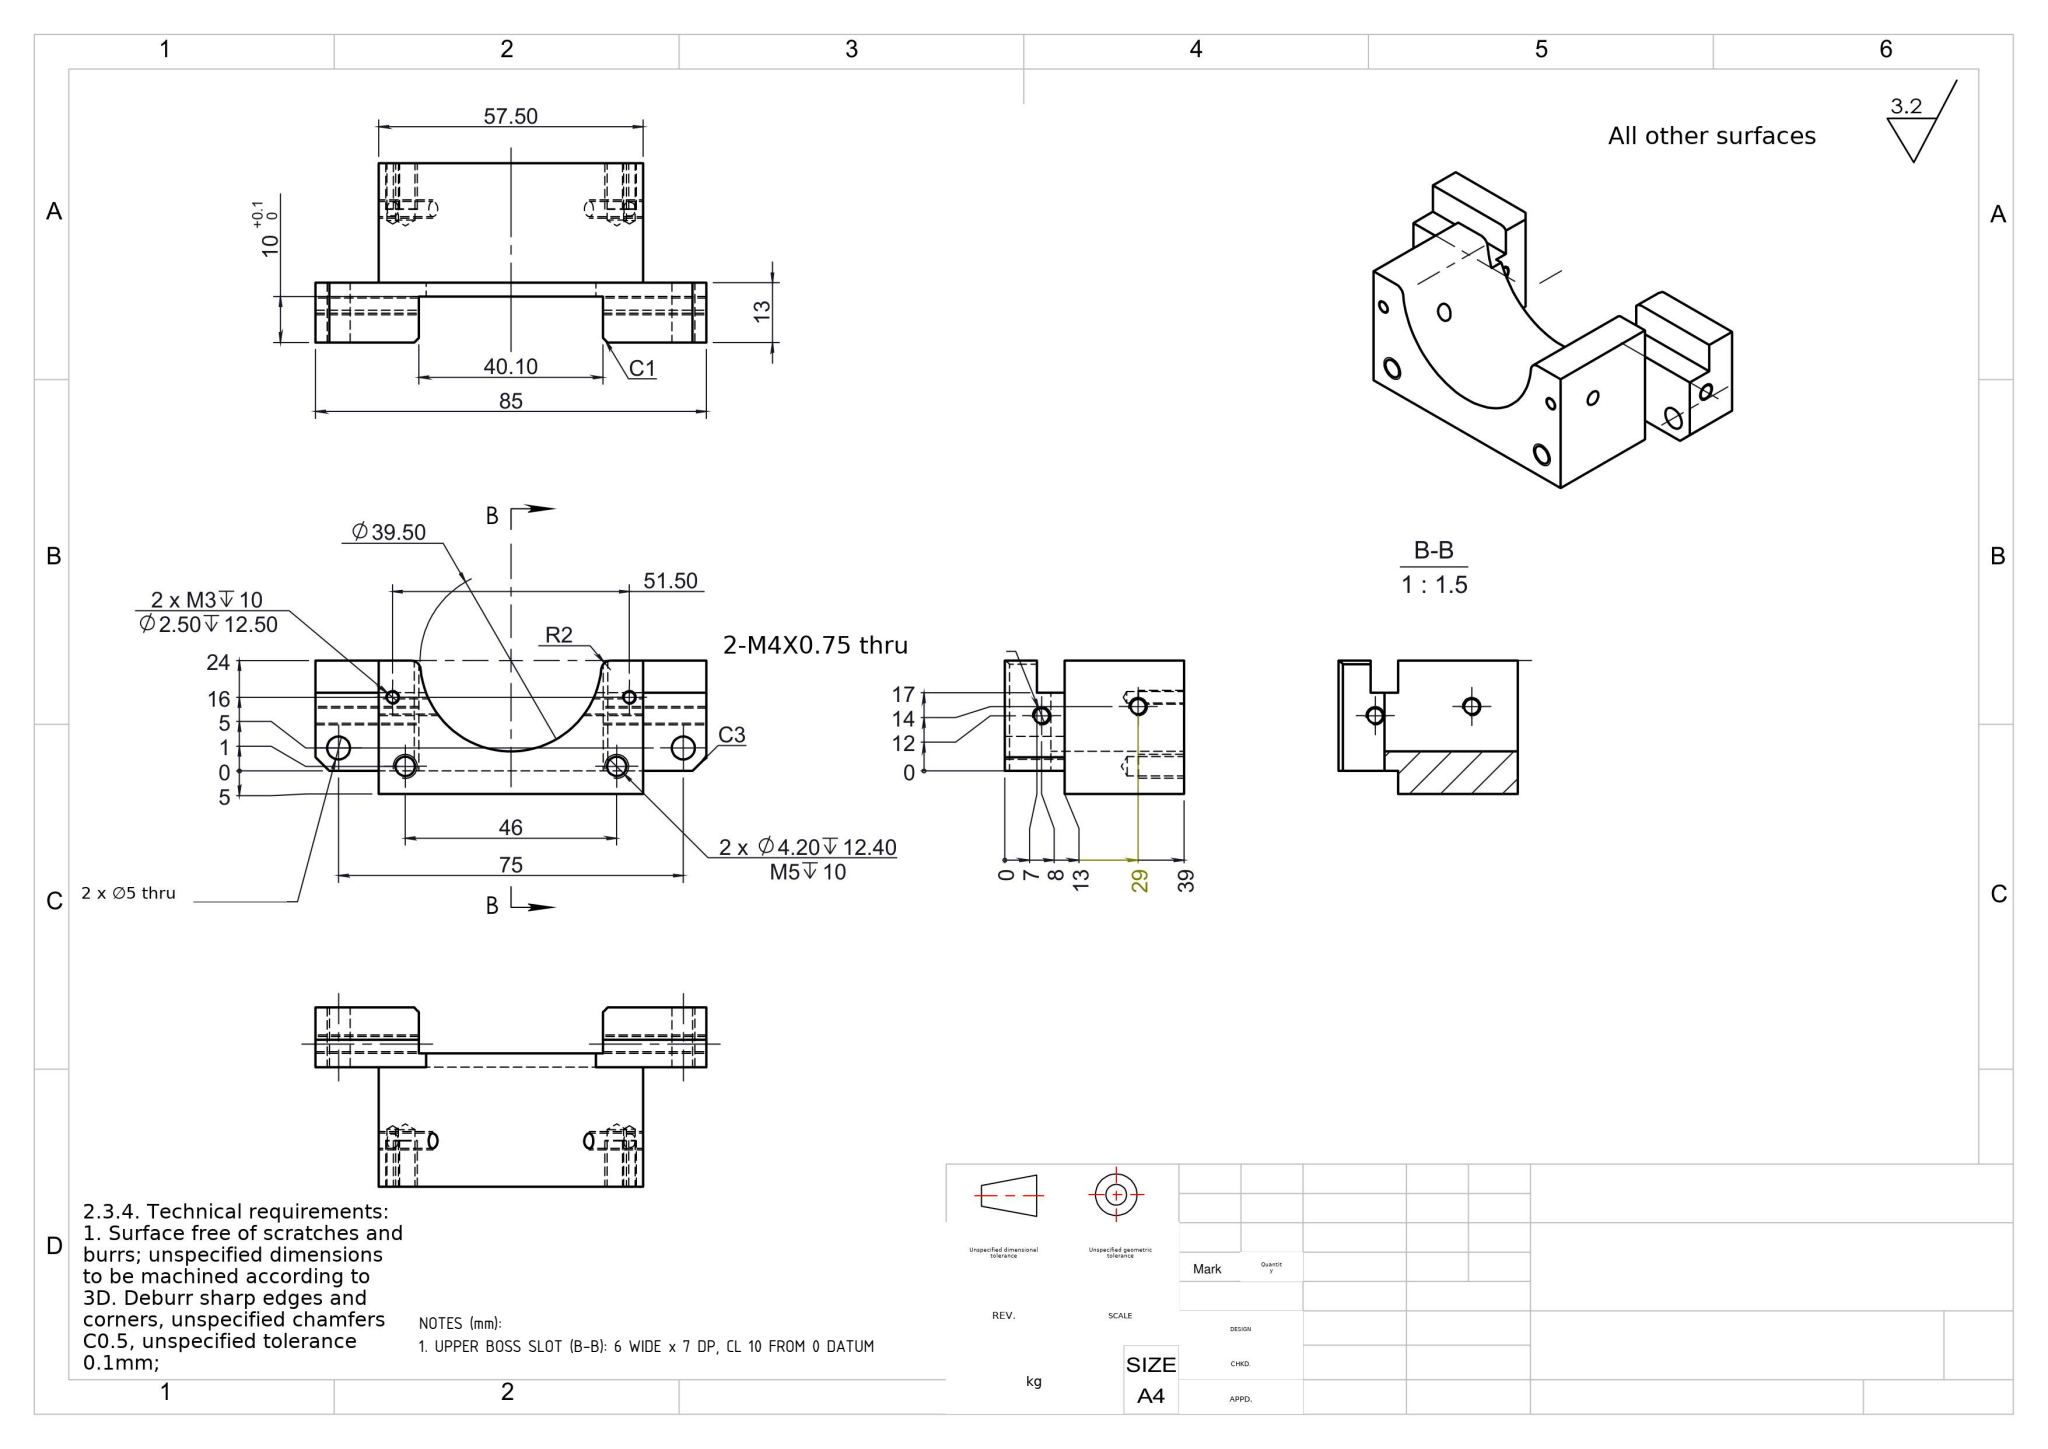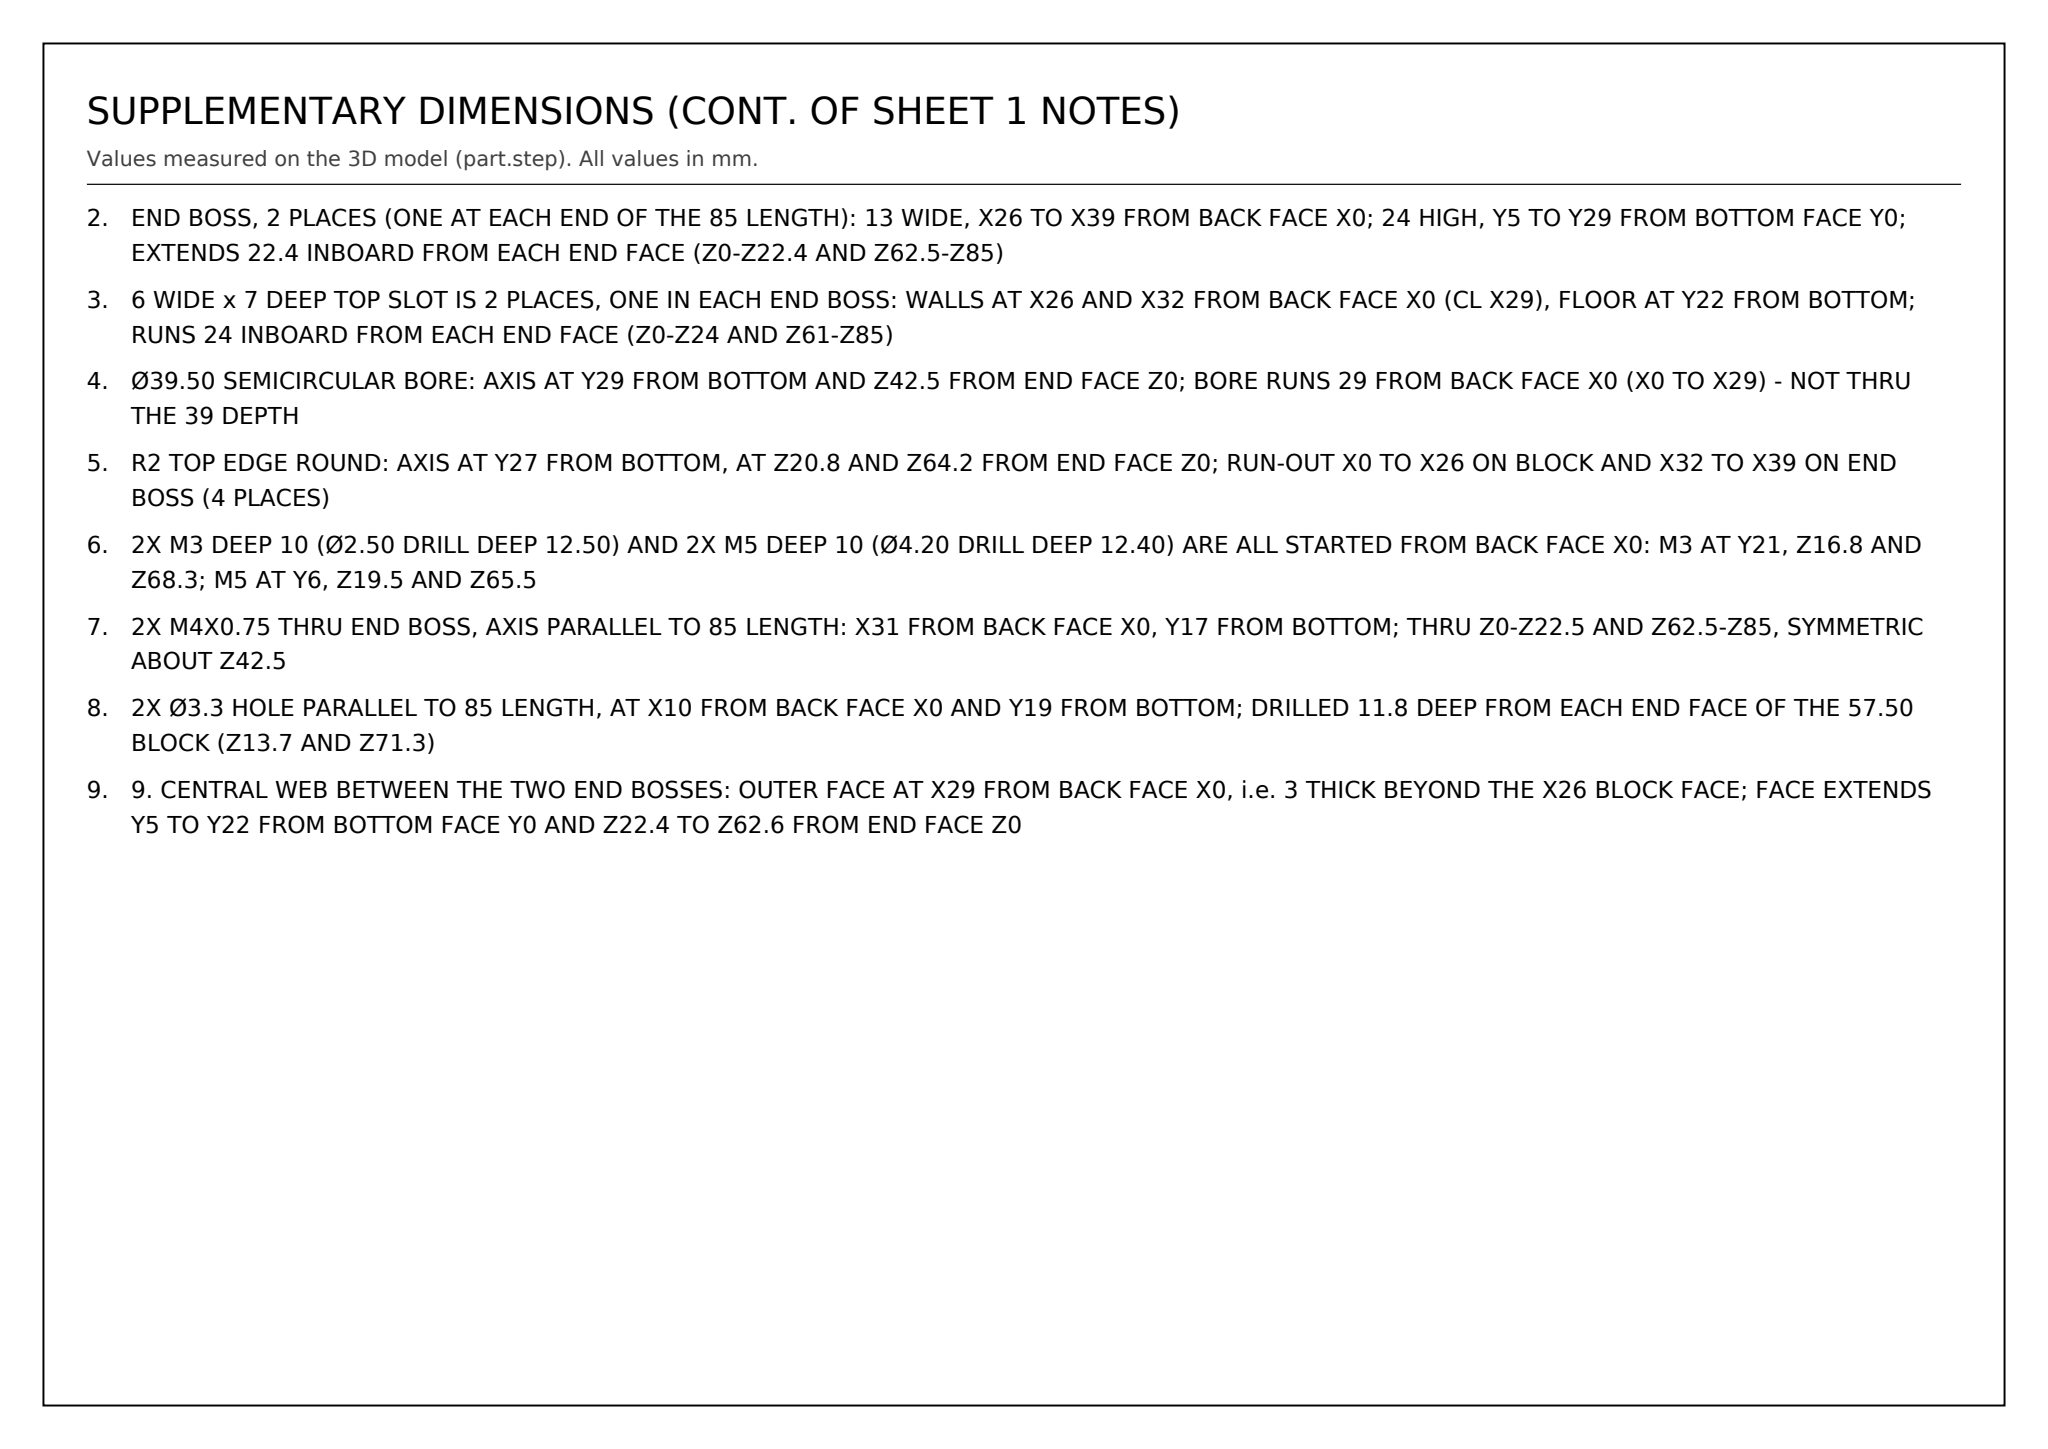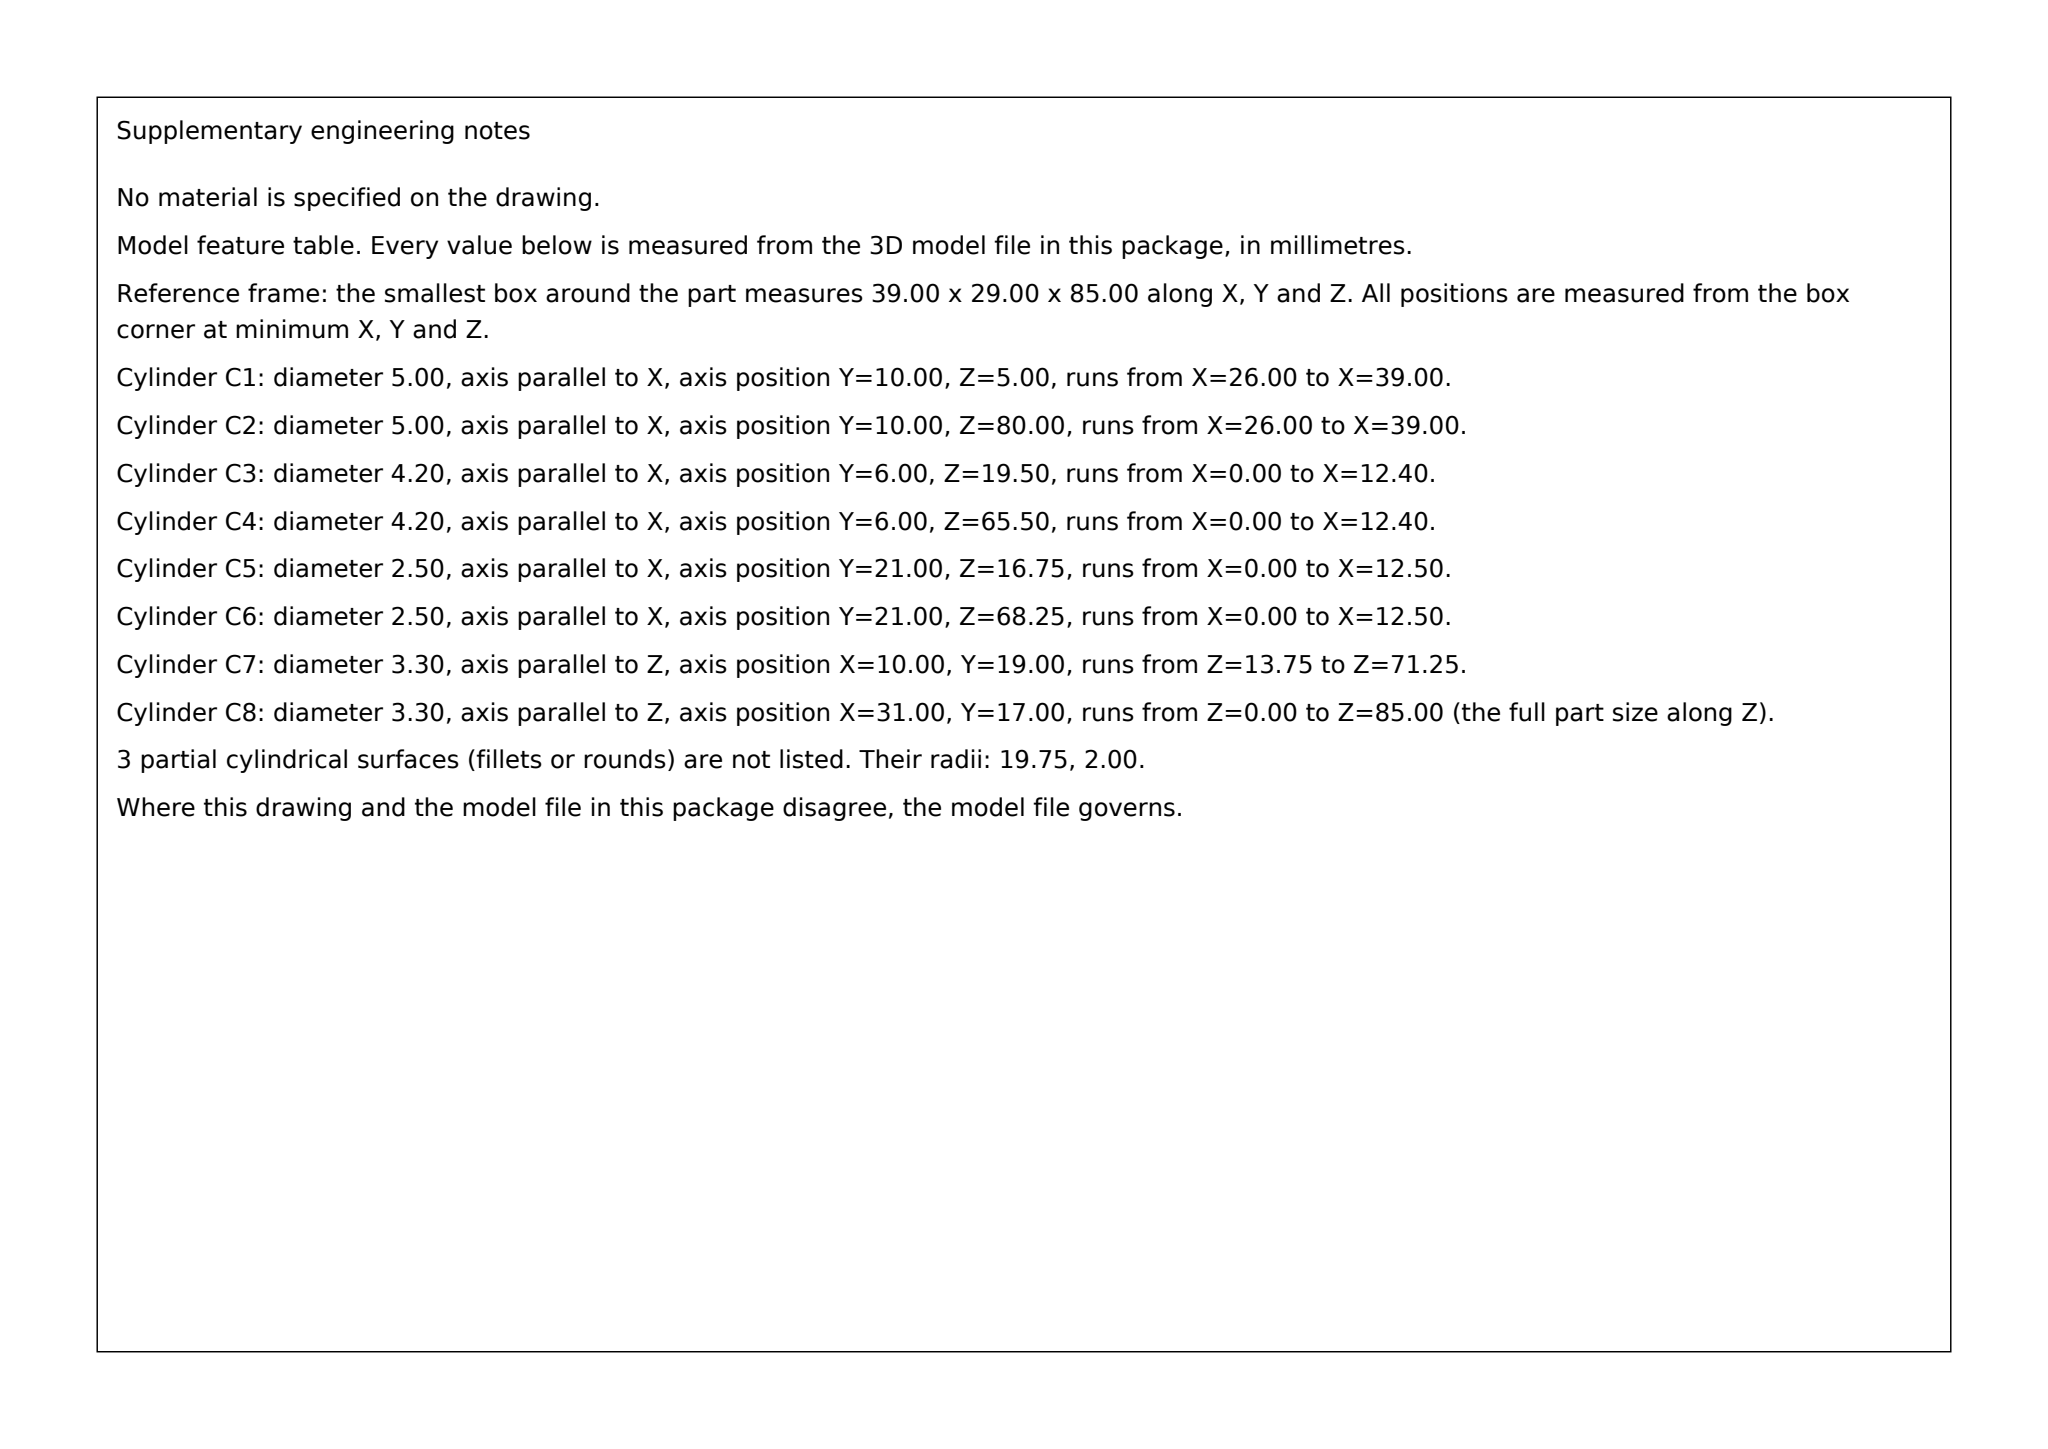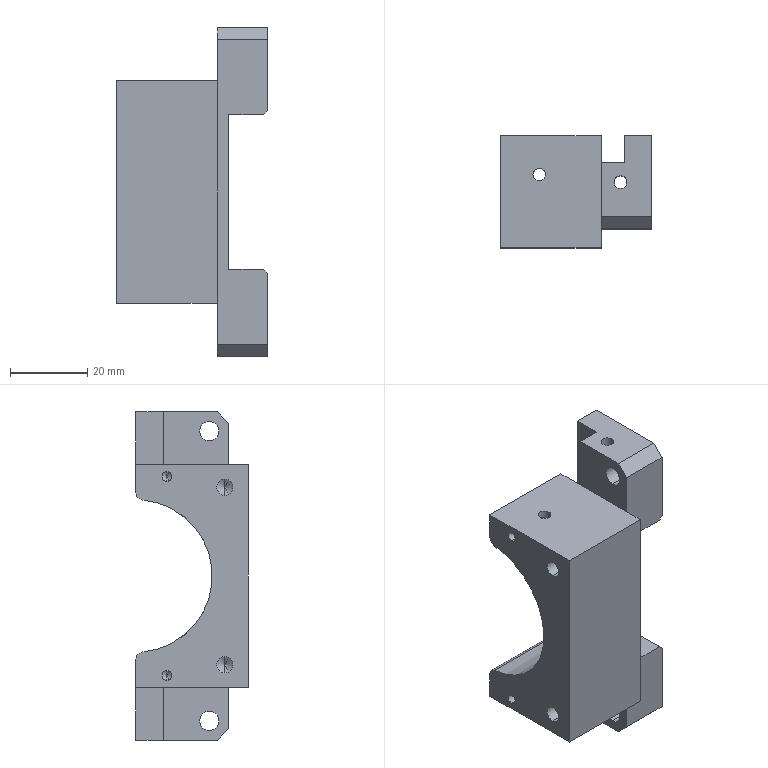Part | SolidWorks | mm | 1 solid | 62 faces | box 39 x 29 x 85 mm | volume 38812 mm3 | plane 29 | cylinder 25 | cone 8 | commonest cylinder face diameters 3.3 x8 4.2 x4 2.5 x4 5 x4 4 x4 39.5 x1
Drawing notes:
UPPER BOSS SLOT (B-B): 6 WIDE x 7 DP, CL 10 FROM 0 DATUM | from the solid: M4 x-holes split into 7 + 26 lg segments over 39 bbox -> gap x=7..13 (6 wide, CL x=10); y-planes 22 (2 slot floors) vs 29 (4 boss tops) -> 7 deep
END BOSS, 2 PLACES (ONE AT EACH END OF THE 85 LENGTH): 13 WIDE, X26 TO X39 FROM BACK FACE X0; 24 HIGH, Y5 TO Y29 FROM BOTTOM FACE Y0; EXTENDS 22.4 INBOARD FROM EACH END FACE (Z0-Z22.4 AND Z62.5-Z85) | from the solid: axis_planes x=26 / x=32 / x=39 (y 5-29), y=5 (x 26-39, z 3-82), z=22.4 and z=62.5 (x 29-38, y 5-28.2)
6 WIDE x 7 DEEP TOP SLOT IS 2 PLACES, ONE IN EACH END BOSS: WALLS AT X26 AND X32 FROM BACK FACE X0 (CL X29), FLOOR AT Y22 FROM BOTTOM; RUNS 24 INBOARD FROM EACH END FACE (Z0-Z24 AND Z61-Z85) | from the solid: axis_planes y=22, extent x 26-32, z 0-24 and z 61-85; planes x=26 and x=32 (y 22-29)
Ø39.50 SEMICIRCULAR BORE: AXIS AT Y29 FROM BOTTOM AND Z42.5 FROM END FACE Z0; BORE RUNS 29 FROM BACK FACE X0 (X0 TO X29) - NOT THRU THE 39 DEPTH | from the solid: cylinder concave arc Ø39.5, axis x, axis_pos y=29 z=42.5, from x 0.0 to 29.0, 169 deg
R2 TOP EDGE ROUND: AXIS AT Y27 FROM BOTTOM, AT Z20.8 AND Z64.2 FROM END FACE Z0; RUN-OUT X0 TO X26 ON BLOCK AND X32 TO X39 ON END BOSS (4 PLACES) | from the solid: convex arcs Ø4.0, axis x, at (y27,z20.8) and (y27,z64.2), from x 0-26 and x 32-39
2X M3 DEEP 10 (Ø2.50 DRILL DEEP 12.50) AND 2X M5 DEEP 10 (Ø4.20 DRILL DEEP 12.40) ARE ALL STARTED FROM BACK FACE X0: M3 AT Y21, Z16.8 AND Z68.3; M5 AT Y6, Z19.5 AND Z65.5 | from the solid: holes Ø2.5 axis x at (y21, z16.8/z68.3) from x0 to 12.5; holes Ø4.2 axis x at (y6, z19.5/z65.5) from x0 to 12.4
2X M4X0.75 THRU END BOSS, AXIS PARALLEL TO 85 LENGTH: X31 FROM BACK FACE X0, Y17 FROM BOTTOM; THRU Z0-Z22.5 AND Z62.5-Z85, SYMMETRIC ABOUT Z42.5 | from the solid: holes Ø3.3 axis z at (x31, y17), from z 0-22.5 and z 62.5-85
2X Ø3.3 HOLE PARALLEL TO 85 LENGTH, AT X10 FROM BACK FACE X0 AND Y19 FROM BOTTOM; DRILLED 11.8 DEEP FROM EACH END FACE OF THE 57.50 BLOCK (Z13.7 AND Z71.3) | from the solid: concave arcs Ø3.3 axis z at (x10, y19), from z 13.7-25.5/26.6 and z 58.4/59.5-71.3; plane z=13.7 area 745 vs 26x29 outline
9. CENTRAL WEB BETWEEN THE TWO END BOSSES: OUTER FACE AT X29 FROM BACK FACE X0, i.e. 3 THICK BEYOND THE X26 BLOCK FACE; FACE EXTENDS Y5 TO Y22 FROM BOTTOM FACE Y0 AND Z22.4 TO Z62.6 FROM END FACE Z0 | from the solid: axis_planes: ['x', 29.0, extent {'y': [5.0, 22.0], 'z': [22.4, 62.6]}, area 340] vs block face ['x', 26.0, ...]